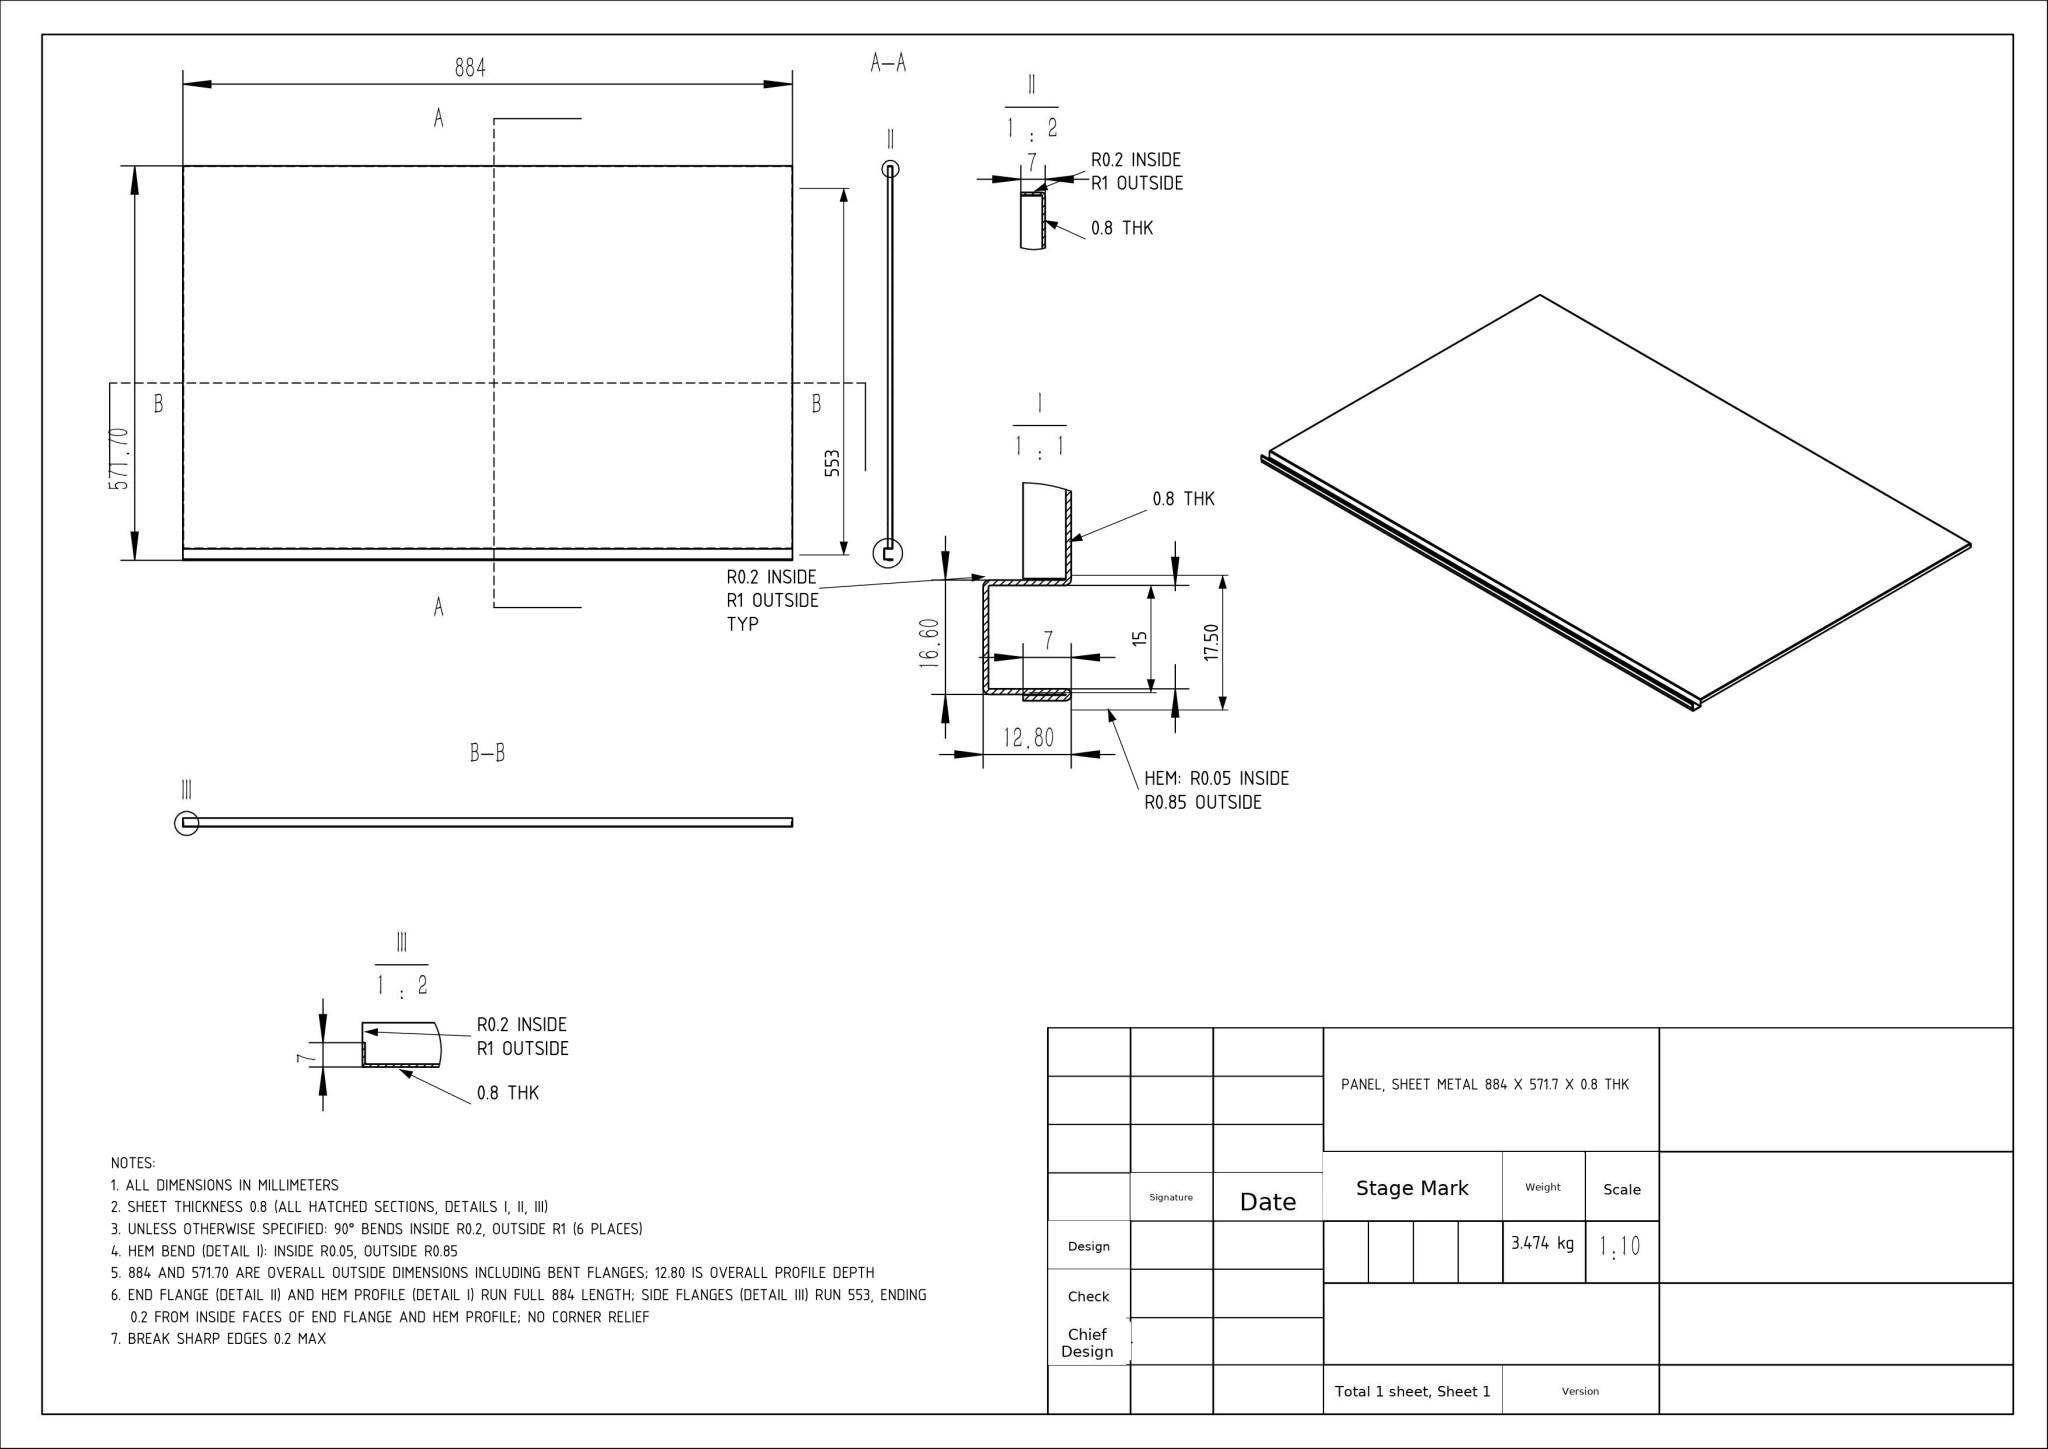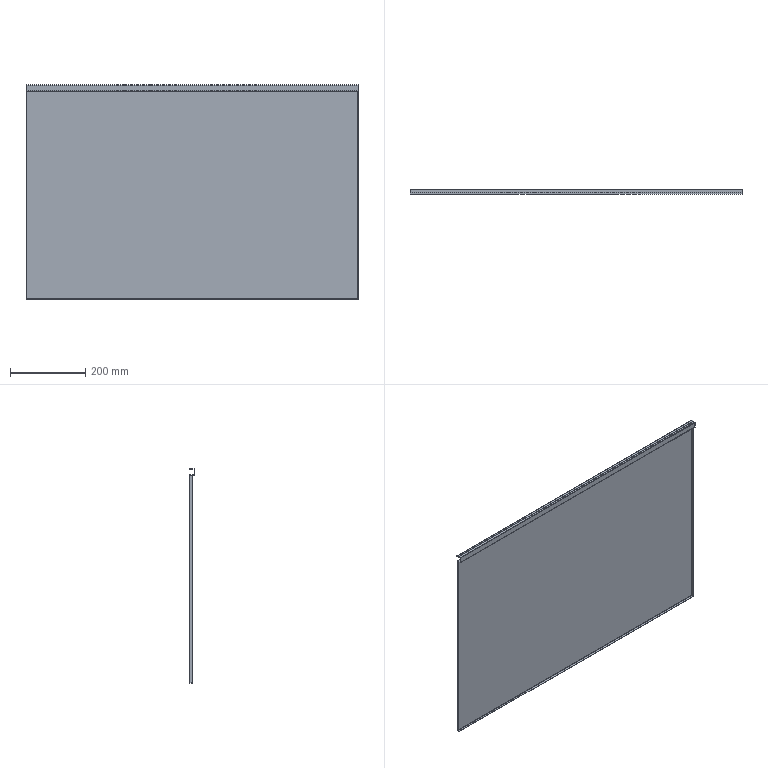Part | NX | mm | 1 solid | 66 faces | box 884 x 12.8 x 571.7 mm | volume 434302 mm3 | plane 52 | cylinder 14 | commonest cylinder face diameters 2 x6 0.4 x6 1.7 x1 0.1 x1